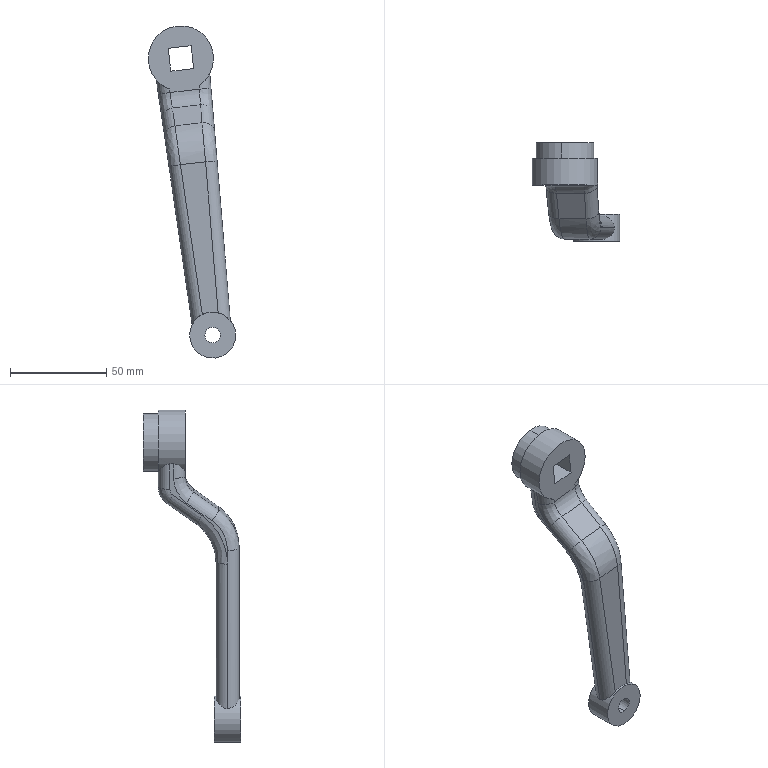Component | SolidWorks | 5-1 | 1 solid | 46 faces | volume 57069 mm3 | cylinder 23 | plane 15 | spline 8 | commonest cylinder face diameters 12 x12 8 x2 24 x2 30 x2 20 x2 50 x2 34 x1